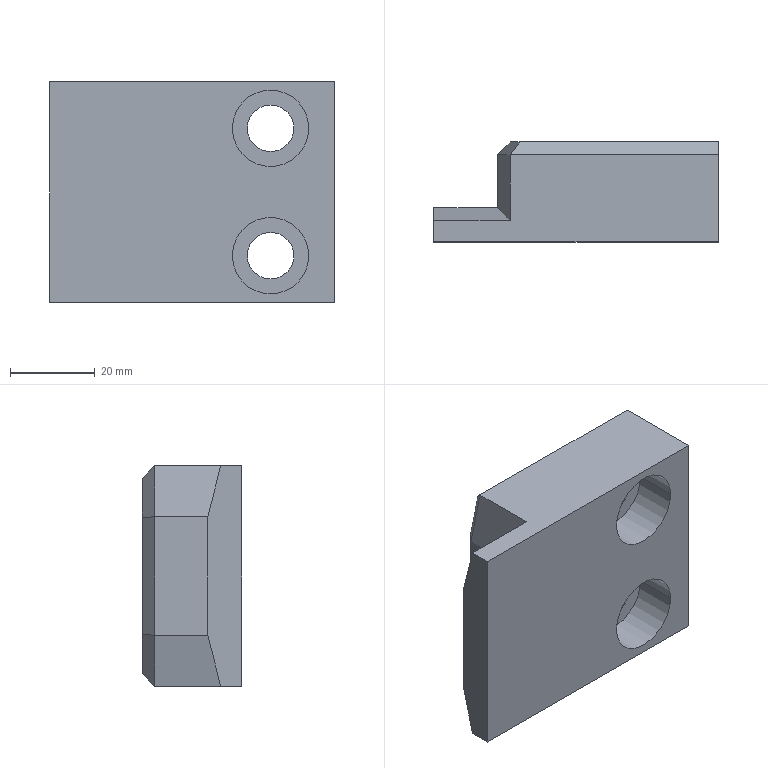Component | SolidWorks | EE8-214-_-_O-2 | 1 solid | 27 faces | box 67 x 23.5 x 52 mm | volume 60297 mm3 | plane 19 | cylinder 8 | commonest cylinder face diameters 18 x4 11 x4
build123d program:
from build123d import *
from OCP.BRepFilletAPI import BRepFilletAPI_MakeChamfer

# Parameters (mm, degrees)
EXTRUDE1_DEPTH                                       = 26
CHAMFER1_SIZE                                        = 3
CHAMFER1_SIZE2                                       = 12
CHAMFER2_SIZE                                        = 12
CHAMFER2_SIZE2                                       = 3
CHAMFER3_SIZE                                        = 3
COUNTERBORE_FOR_M10_SOCKET_HEAD_CAP_SCRE_D           = 11
COUNTERBORE_FOR_M10_SOCKET_HEAD_CAP_SCRE_CBORE_D     = 18
COUNTERBORE_FOR_M10_SOCKET_HEAD_CAP_SCRE_CBORE_DEPTH = 10


with BuildPart() as part:
    # Sketch1 → Extrude1 (new, symmetric)
    with BuildSketch(Plane(origin=(0, 0, 0), x_dir=(0, 0, -1), z_dir=(1, 0, 0))):
        Polygon((0, 0), (0, 23.5), (-52, 23.5), (-52, 8), (-67, 8), (-67, 0), align=None)
    extrude(amount=EXTRUDE1_DEPTH, both=True)

    # Chamfer1
    chamfer1_edges = [part.edges().sort_by_distance(p)[0] for p in [
        (-26, 8, 59.5),
        (-26, 15.75, 52),
    ]]
    chamfer1_side = [part.faces().sort_by_distance(p)[0] for p in [
        (-26, 11.057, 28.996),
    ]]
    chamfer(chamfer1_edges, length=CHAMFER1_SIZE, length2=CHAMFER1_SIZE2, reference=chamfer1_side[0])

    # Chamfer2: one chamfer whose edges measure the first distance from different faces: ONE call of the kernel's chamfer builder (chamfer() names one face for all edges)
    chamfer2_edges_1 = [part.edges().sort_by_distance(p)[0] for p in [
        (26, 15.75, 52),
    ]]
    chamfer2_side_1 = [part.faces().sort_by_distance(p)[0] for p in [
        (6, 15.75, 52),
    ]]
    chamfer2_edges_2 = [part.edges().sort_by_distance(p)[0] for p in [
        (26, 8, 59.5),
    ]]
    chamfer2_side_2 = [part.faces().sort_by_distance(p)[0] for p in [
        (6, 8, 59.5),
    ]]
    chamfer2 = BRepFilletAPI_MakeChamfer(part.part.solid().wrapped)
    for e in chamfer2_edges_1:
        chamfer2.Add(CHAMFER2_SIZE, CHAMFER2_SIZE2, e.wrapped, chamfer2_side_1[0].wrapped)  # the first distance lies on this face
    for e in chamfer2_edges_2:
        chamfer2.Add(CHAMFER2_SIZE, CHAMFER2_SIZE2, e.wrapped, chamfer2_side_2[0].wrapped)  # the first distance lies on this face
    add(Compound.cast(chamfer2.Shape()), mode=Mode.REPLACE)

    # Chamfer3
    chamfer3_edges = [part.edges().sort_by_distance(p)[0] for p in [
        (26, 23.5, 24.5),
        (-20, 23.5, 50.5),
        (0, 23.5, 52),
        (20, 23.5, 50.5),
        (-26, 23.5, 24.5),
    ]]
    chamfer(chamfer3_edges, length=CHAMFER3_SIZE)

    # Counterbore for M10 Socket Head Cap Scre (through all)
    with Locations(Plane.XZ):
        with Locations((15, 15), (-15, 15)):
            CounterBoreHole(COUNTERBORE_FOR_M10_SOCKET_HEAD_CAP_SCRE_D / 2, COUNTERBORE_FOR_M10_SOCKET_HEAD_CAP_SCRE_CBORE_D / 2, COUNTERBORE_FOR_M10_SOCKET_HEAD_CAP_SCRE_CBORE_DEPTH)


solid = part.part

# Placed as in the assembly
solid = solid.moved(Location((15, -23.5, -230), (0, -90, 0)))
STEP:
#1=CARTESIAN_POINT('',(-0.3543,-0.5315,-9.646));
#2=VERTEX_POINT('',#1);
#3=CARTESIAN_POINT('',(0.3543,-0.5315,-9.646));
#4=VERTEX_POINT('',#3);
#5=CARTESIAN_POINT('',(-0.,-0.5315,-9.646));
#6=DIRECTION('',(0.,-1.,0.));
#7=DIRECTION('',(1.,0.,-0.));
#8=AXIS2_PLACEMENT_3D('',#5,#6,#7);
#9=CIRCLE('',#8,0.3543);
#10=EDGE_CURVE('',#2,#4,#9,.T.);
#11=ORIENTED_EDGE('',*,*,#10,.F.);
#12=CARTESIAN_POINT('',(-0.3543,-0.9252,-9.646));
#13=VERTEX_POINT('',#12);
#14=CARTESIAN_POINT('',(-0.3543,-0.9252,-9.646));
#15=DIRECTION('',(0.,-1.,0.));
#16=VECTOR('',#15,39.37);
#17=LINE('',#14,#16);
#18=EDGE_CURVE('',#2,#13,#17,.T.);
#19=ORIENTED_EDGE('',*,*,#18,.T.);
#20=CARTESIAN_POINT('',(0.3543,-0.9252,-9.646));
#21=VERTEX_POINT('',#20);
#22=CARTESIAN_POINT('',(-0.,-0.9252,-9.646));
#23=DIRECTION('',(0.,-1.,0.));
#24=DIRECTION('',(1.,0.,-0.));
#25=AXIS2_PLACEMENT_3D('',#22,#23,#24);
#26=CIRCLE('',#25,0.3543);
#27=EDGE_CURVE('',#13,#21,#26,.T.);
#28=ORIENTED_EDGE('',*,*,#27,.T.);
#29=CARTESIAN_POINT('',(0.3543,-0.9252,-9.646));
#30=DIRECTION('',(0.,-1.,0.));
#31=VECTOR('',#30,39.37);
#32=LINE('',#29,#31);
#33=EDGE_CURVE('',#4,#21,#32,.T.);
#34=ORIENTED_EDGE('',*,*,#33,.F.);
#35=EDGE_LOOP('',(#11,#19,#28,#34));
#36=FACE_OUTER_BOUND('',#35,.T.);
#37=CARTESIAN_POINT('',(-0.,-0.9252,-9.646));
#38=DIRECTION('',(0.,-1.,0.));
#39=DIRECTION('',(1.,0.,-0.));
#40=AXIS2_PLACEMENT_3D('',#37,#38,#39);
#41=CYLINDRICAL_SURFACE('',#40,0.3543);
#42=ADVANCED_FACE('',(#36),#41,.F.);
#43=CARTESIAN_POINT('',(-0.2165,0.,-9.646));
#44=VERTEX_POINT('',#43);
#45=CARTESIAN_POINT('',(0.2165,0.,-9.646));
#46=VERTEX_POINT('',#45);
#47=CARTESIAN_POINT('',(-0.,0.,-9.646));
#48=DIRECTION('',(0.,-1.,0.));
#49=DIRECTION('',(1.,0.,-0.));
#50=AXIS2_PLACEMENT_3D('',#47,#48,#49);
#51=CIRCLE('',#50,0.2165);
#52=EDGE_CURVE('',#44,#46,#51,.T.);
#53=ORIENTED_EDGE('',*,*,#52,.F.);
#54=CARTESIAN_POINT('',(-0.2165,-0.5315,-9.646));
#55=VERTEX_POINT('',#54);
#56=CARTESIAN_POINT('',(-0.2165,-0.9252,-9.646));
#57=DIRECTION('',(0.,-1.,0.));
#58=VECTOR('',#57,39.37);
#59=LINE('',#56,#58);
#60=EDGE_CURVE('',#44,#55,#59,.T.);
#61=ORIENTED_EDGE('',*,*,#60,.T.);
#62=CARTESIAN_POINT('',(0.2165,-0.5315,-9.646));
#63=VERTEX_POINT('',#62);
#64=CARTESIAN_POINT('',(-0.,-0.5315,-9.646));
#65=DIRECTION('',(0.,-1.,0.));
#66=DIRECTION('',(1.,0.,-0.));
#67=AXIS2_PLACEMENT_3D('',#64,#65,#66);
#68=CIRCLE('',#67,0.2165);
#69=EDGE_CURVE('',#55,#63,#68,.T.);
#70=ORIENTED_EDGE('',*,*,#69,.T.);
#71=CARTESIAN_POINT('',(0.2165,-0.9252,-9.646));
#72=DIRECTION('',(0.,-1.,0.));
#73=VECTOR('',#72,39.37);
#74=LINE('',#71,#73);
#75=EDGE_CURVE('',#46,#63,#74,.T.);
#76=ORIENTED_EDGE('',*,*,#75,.F.);
#77=EDGE_LOOP('',(#53,#61,#70,#76));
#78=FACE_OUTER_BOUND('',#77,.T.);
#79=CARTESIAN_POINT('',(-0.,-0.9252,-9.646));
#80=DIRECTION('',(0.,-1.,0.));
#81=DIRECTION('',(1.,0.,-0.));
#82=AXIS2_PLACEMENT_3D('',#79,#80,#81);
#83=CYLINDRICAL_SURFACE('',#82,0.2165);
#84=ADVANCED_FACE('',(#78),#83,.F.);
#85=CARTESIAN_POINT('',(-0.3543,-0.5315,-8.465));
#86=VERTEX_POINT('',#85);
#87=CARTESIAN_POINT('',(0.3543,-0.5315,-8.465));
#88=VERTEX_POINT('',#87);
#89=CARTESIAN_POINT('',(-0.,-0.5315,-8.465));
#90=DIRECTION('',(0.,-1.,0.));
#91=DIRECTION('',(1.,0.,-0.));
#92=AXIS2_PLACEMENT_3D('',#89,#90,#91);
#93=CIRCLE('',#92,0.3543);
#94=EDGE_CURVE('',#86,#88,#93,.T.);
#95=ORIENTED_EDGE('',*,*,#94,.F.);
#96=CARTESIAN_POINT('',(-0.3543,-0.9252,-8.465));
#97=VERTEX_POINT('',#96);
#98=CARTESIAN_POINT('',(-0.3543,-0.9252,-8.465));
#99=DIRECTION('',(0.,-1.,0.));
#100=VECTOR('',#99,39.37);
#101=LINE('',#98,#100);
#102=EDGE_CURVE('',#86,#97,#101,.T.);
#103=ORIENTED_EDGE('',*,*,#102,.T.);
#104=CARTESIAN_POINT('',(0.3543,-0.9252,-8.465));
#105=VERTEX_POINT('',#104);
#106=CARTESIAN_POINT('',(-0.,-0.9252,-8.465));
#107=DIRECTION('',(0.,-1.,0.));
#108=DIRECTION('',(1.,0.,-0.));
#109=AXIS2_PLACEMENT_3D('',#106,#107,#108);
#110=CIRCLE('',#109,0.3543);
#111=EDGE_CURVE('',#97,#105,#110,.T.);
#112=ORIENTED_EDGE('',*,*,#111,.T.);
#113=CARTESIAN_POINT('',(0.3543,-0.9252,-8.465));
#114=DIRECTION('',(0.,-1.,0.));
#115=VECTOR('',#114,39.37);
#116=LINE('',#113,#115);
#117=EDGE_CURVE('',#88,#105,#116,.T.);
#118=ORIENTED_EDGE('',*,*,#117,.F.);
#119=EDGE_LOOP('',(#95,#103,#112,#118));
#120=FACE_OUTER_BOUND('',#119,.T.);
#121=CARTESIAN_POINT('',(-0.,-0.9252,-8.465));
#122=DIRECTION('',(0.,-1.,0.));
#123=DIRECTION('',(1.,0.,-0.));
#124=AXIS2_PLACEMENT_3D('',#121,#122,#123);
#125=CYLINDRICAL_SURFACE('',#124,0.3543);
#126=ADVANCED_FACE('',(#120),#125,.F.);
#127=CARTESIAN_POINT('',(-0.2165,0.,-8.465));
#128=VERTEX_POINT('',#127);
#129=CARTESIAN_POINT('',(0.2165,0.,-8.465));
#130=VERTEX_POINT('',#129);
#131=CARTESIAN_POINT('',(-0.,0.,-8.465));
#132=DIRECTION('',(0.,-1.,0.));
#133=DIRECTION('',(1.,0.,-0.));
#134=AXIS2_PLACEMENT_3D('',#131,#132,#133);
#135=CIRCLE('',#134,0.2165);
#136=EDGE_CURVE('',#128,#130,#135,.T.);
#137=ORIENTED_EDGE('',*,*,#136,.F.);
#138=CARTESIAN_POINT('',(-0.2165,-0.5315,-8.465));
#139=VERTEX_POINT('',#138);
#140=CARTESIAN_POINT('',(-0.2165,-0.9252,-8.465));
#141=DIRECTION('',(0.,-1.,0.));
#142=VECTOR('',#141,39.37);
#143=LINE('',#140,#142);
#144=EDGE_CURVE('',#128,#139,#143,.T.);
#145=ORIENTED_EDGE('',*,*,#144,.T.);
#146=CARTESIAN_POINT('',(0.2165,-0.5315,-8.465));
#147=VERTEX_POINT('',#146);
#148=CARTESIAN_POINT('',(-0.,-0.5315,-8.465));
#149=DIRECTION('',(0.,-1.,0.));
#150=DIRECTION('',(1.,0.,-0.));
#151=AXIS2_PLACEMENT_3D('',#148,#149,#150);
#152=CIRCLE('',#151,0.2165);
#153=EDGE_CURVE('',#139,#147,#152,.T.);
#154=ORIENTED_EDGE('',*,*,#153,.T.);
#155=CARTESIAN_POINT('',(0.2165,-0.9252,-8.465));
#156=DIRECTION('',(0.,-1.,0.));
#157=VECTOR('',#156,39.37);
#158=LINE('',#155,#157);
#159=EDGE_CURVE('',#130,#147,#158,.T.);
#160=ORIENTED_EDGE('',*,*,#159,.F.);
#161=EDGE_LOOP('',(#137,#145,#154,#160));
#162=FACE_OUTER_BOUND('',#161,.T.);
#163=CARTESIAN_POINT('',(-0.,-0.9252,-8.465));
#164=DIRECTION('',(0.,-1.,0.));
#165=DIRECTION('',(1.,0.,-0.));
#166=AXIS2_PLACEMENT_3D('',#163,#164,#165);
#167=CYLINDRICAL_SURFACE('',#166,0.2165);
#168=ADVANCED_FACE('',(#162),#167,.F.);
#169=CARTESIAN_POINT('',(-0.,-0.9252,-9.646));
#170=DIRECTION('',(0.,-1.,0.));
#171=DIRECTION('',(1.,0.,-0.));
#172=AXIS2_PLACEMENT_3D('',#169,#170,#171);
#173=CIRCLE('',#172,0.3543);
#174=EDGE_CURVE('',#21,#13,#173,.T.);
#175=ORIENTED_EDGE('',*,*,#174,.F.);
#176=ORIENTED_EDGE('',*,*,#27,.F.);
#177=EDGE_LOOP('',(#175,#176));
#178=FACE_BOUND('',#177,.T.);
#179=CARTESIAN_POINT('',(-2.047,-0.9252,-10.079));
#180=VERTEX_POINT('',#179);
#181=CARTESIAN_POINT('',(0.5906,-0.9252,-10.079));
#182=VERTEX_POINT('',#181);
#183=CARTESIAN_POINT('',(-2.047,-0.9252,-10.079));
#184=DIRECTION('',(1.,0.,-0.));
#185=VECTOR('',#184,39.37);
#186=LINE('',#183,#185);
#187=EDGE_CURVE('',#180,#182,#186,.T.);
#188=ORIENTED_EDGE('',*,*,#187,.T.);
#189=CARTESIAN_POINT('',(0.5906,-0.9252,-8.031));
#190=VERTEX_POINT('',#189);
#191=CARTESIAN_POINT('',(0.5906,-0.9252,-8.031));
#192=DIRECTION('',(-0.,0.,-1.));
#193=VECTOR('',#192,39.37);
#194=LINE('',#191,#193);
#195=EDGE_CURVE('',#190,#182,#194,.T.);
#196=ORIENTED_EDGE('',*,*,#195,.F.);
#197=CARTESIAN_POINT('',(-2.047,-0.9252,-8.031));
#198=VERTEX_POINT('',#197);
#199=CARTESIAN_POINT('',(-2.047,-0.9252,-8.031));
#200=DIRECTION('',(1.,0.,-0.));
#201=VECTOR('',#200,39.37);
#202=LINE('',#199,#201);
#203=EDGE_CURVE('',#198,#190,#202,.T.);
#204=ORIENTED_EDGE('',*,*,#203,.F.);
#205=CARTESIAN_POINT('',(-2.047,-0.9252,-8.031));
#206=DIRECTION('',(-0.,0.,-1.));
#207=VECTOR('',#206,39.37);
#208=LINE('',#205,#207);
#209=EDGE_CURVE('',#198,#180,#208,.T.);
#210=ORIENTED_EDGE('',*,*,#209,.T.);
#211=EDGE_LOOP('',(#188,#196,#204,#210));
#212=FACE_OUTER_BOUND('',#211,.T.);
#213=CARTESIAN_POINT('',(-0.,-0.9252,-8.465));
#214=DIRECTION('',(0.,-1.,0.));
#215=DIRECTION('',(1.,0.,-0.));
#216=AXIS2_PLACEMENT_3D('',#213,#214,#215);
#217=CIRCLE('',#216,0.3543);
#218=EDGE_CURVE('',#105,#97,#217,.T.);
#219=ORIENTED_EDGE('',*,*,#218,.F.);
#220=ORIENTED_EDGE('',*,*,#111,.F.);
#221=EDGE_LOOP('',(#219,#220));
#222=FACE_BOUND('',#221,.T.);
#223=CARTESIAN_POINT('',(-2.047,-0.9252,-8.031));
#224=DIRECTION('',(0.,1.,0.));
#225=DIRECTION('',(-1.,0.,0.));
#226=AXIS2_PLACEMENT_3D('',#223,#224,#225);
#227=PLANE('',#226);
#228=ADVANCED_FACE('',(#178,#212,#222),#227,.F.);
#229=CARTESIAN_POINT('',(0.5906,-0.1181,-10.079));
#230=VERTEX_POINT('',#229);
#231=CARTESIAN_POINT('',(0.5906,-0.9252,-10.079));
#232=DIRECTION('',(0.,1.,0.));
#233=VECTOR('',#232,39.37);
#234=LINE('',#231,#233);
#235=EDGE_CURVE('',#182,#230,#234,.T.);
#236=ORIENTED_EDGE('',*,*,#235,.T.);
#237=CARTESIAN_POINT('',(0.5906,0.,-9.961));
#238=VERTEX_POINT('',#237);
#239=CARTESIAN_POINT('',(0.5906,0.,-9.961));
#240=DIRECTION('',(0.,0.7071,0.7071));
#241=VECTOR('',#240,39.37);
#242=LINE('',#239,#241);
#243=EDGE_CURVE('',#230,#238,#242,.T.);
#244=ORIENTED_EDGE('',*,*,#243,.T.);
#245=CARTESIAN_POINT('',(0.5906,0.,-8.15));
#246=VERTEX_POINT('',#245);
#247=CARTESIAN_POINT('',(0.5906,0.,-8.031));
#248=DIRECTION('',(-0.,0.,-1.));
#249=VECTOR('',#248,39.37);
#250=LINE('',#247,#249);
#251=EDGE_CURVE('',#246,#238,#250,.T.);
#252=ORIENTED_EDGE('',*,*,#251,.F.);
#253=CARTESIAN_POINT('',(0.5906,-0.1181,-8.031));
#254=VERTEX_POINT('',#253);
#255=CARTESIAN_POINT('',(0.5906,-0.1181,-8.031));
#256=DIRECTION('',(0.,-0.7071,0.7071));
#257=VECTOR('',#256,39.37);
#258=LINE('',#255,#257);
#259=EDGE_CURVE('',#246,#254,#258,.T.);
#260=ORIENTED_EDGE('',*,*,#259,.T.);
#261=CARTESIAN_POINT('',(0.5906,-0.9252,-8.031));
#262=DIRECTION('',(0.,1.,0.));
#263=VECTOR('',#262,39.37);
#264=LINE('',#261,#263);
#265=EDGE_CURVE('',#190,#254,#264,.T.);
#266=ORIENTED_EDGE('',*,*,#265,.F.);
#267=ORIENTED_EDGE('',*,*,#195,.T.);
#268=EDGE_LOOP('',(#236,#244,#252,#260,#266,#267));
#269=FACE_OUTER_BOUND('',#268,.T.);
#270=CARTESIAN_POINT('',(0.5906,-0.9252,-8.031));
#271=DIRECTION('',(-1.,0.,0.));
#272=DIRECTION('',(0.,0.,1.));
#273=AXIS2_PLACEMENT_3D('',#270,#271,#272);
#274=PLANE('',#273);
#275=ADVANCED_FACE('',(#269),#274,.F.);
#276=CARTESIAN_POINT('',(-0.,0.,-9.646));
#277=DIRECTION('',(0.,-1.,0.));
#278=DIRECTION('',(1.,0.,-0.));
#279=AXIS2_PLACEMENT_3D('',#276,#277,#278);
#280=CIRCLE('',#279,0.2165);
#281=EDGE_CURVE('',#46,#44,#280,.T.);
#282=ORIENTED_EDGE('',*,*,#281,.T.);
#283=ORIENTED_EDGE('',*,*,#52,.T.);
#284=EDGE_LOOP('',(#282,#283));
#285=FACE_BOUND('',#284,.T.);
#286=CARTESIAN_POINT('',(-0.,0.,-8.465));
#287=DIRECTION('',(0.,-1.,0.));
#288=DIRECTION('',(1.,0.,-0.));
#289=AXIS2_PLACEMENT_3D('',#286,#287,#288);
#290=CIRCLE('',#289,0.2165);
#291=EDGE_CURVE('',#130,#128,#290,.T.);
#292=ORIENTED_EDGE('',*,*,#291,.T.);
#293=ORIENTED_EDGE('',*,*,#136,.T.);
#294=EDGE_LOOP('',(#292,#293));
#295=FACE_BOUND('',#294,.T.);
#296=ORIENTED_EDGE('',*,*,#251,.T.);
#297=CARTESIAN_POINT('',(-1.246,-0.,-9.961));
#298=VERTEX_POINT('',#297);
#299=CARTESIAN_POINT('',(0.5906,0.,-9.961));
#300=DIRECTION('',(-1.,-0.,0.));
#301=VECTOR('',#300,39.37);
#302=LINE('',#299,#301);
#303=EDGE_CURVE('',#238,#298,#302,.T.);
#304=ORIENTED_EDGE('',*,*,#303,.T.);
#305=CARTESIAN_POINT('',(-1.339,-0.,-9.592));
#306=VERTEX_POINT('',#305);
#307=CARTESIAN_POINT('',(-1.342,-0.,-9.578));
#308=DIRECTION('',(-0.2425,-0.,0.9701));
#309=VECTOR('',#308,39.37);
#310=LINE('',#307,#309);
#311=EDGE_CURVE('',#298,#306,#310,.T.);
#312=ORIENTED_EDGE('',*,*,#311,.T.);
#313=CARTESIAN_POINT('',(-1.339,-0.,-8.518));
#314=VERTEX_POINT('',#313);
#315=CARTESIAN_POINT('',(-1.339,-0.,-8.031));
#316=DIRECTION('',(0.,0.,1.));
#317=VECTOR('',#316,39.37);
#318=LINE('',#315,#317);
#319=EDGE_CURVE('',#306,#314,#318,.T.);
#320=ORIENTED_EDGE('',*,*,#319,.T.);
#321=CARTESIAN_POINT('',(-1.246,-0.,-8.15));
#322=VERTEX_POINT('',#321);
#323=CARTESIAN_POINT('',(-1.224,-0.,-8.06));
#324=DIRECTION('',(0.2425,0.,0.9701));
#325=VECTOR('',#324,39.37);
#326=LINE('',#323,#325);
#327=EDGE_CURVE('',#314,#322,#326,.T.);
#328=ORIENTED_EDGE('',*,*,#327,.T.);
#329=CARTESIAN_POINT('',(0.5906,0.,-8.15));
#330=DIRECTION('',(1.,0.,-0.));
#331=VECTOR('',#330,39.37);
#332=LINE('',#329,#331);
#333=EDGE_CURVE('',#322,#246,#332,.T.);
#334=ORIENTED_EDGE('',*,*,#333,.T.);
#335=EDGE_LOOP('',(#296,#304,#312,#320,#328,#334));
#336=FACE_OUTER_BOUND('',#335,.T.);
#337=CARTESIAN_POINT('',(0.5906,0.,-8.031));
#338=DIRECTION('',(0.,-1.,-0.));
#339=DIRECTION('',(1.,0.,-0.));
#340=AXIS2_PLACEMENT_3D('',#337,#338,#339);
#341=PLANE('',#340);
#342=ADVANCED_FACE('',(#285,#295,#336),#341,.F.);
#343=CARTESIAN_POINT('',(-1.457,-0.6102,-8.504));
#344=VERTEX_POINT('',#343);
#345=CARTESIAN_POINT('',(-1.457,-0.1181,-8.504));
#346=VERTEX_POINT('',#345);
#347=CARTESIAN_POINT('',(-1.457,-0.,-8.504));
#348=DIRECTION('',(-0.,1.,0.));
#349=VECTOR('',#348,39.37);
#350=LINE('',#347,#349);
#351=EDGE_CURVE('',#344,#346,#350,.T.);
#352=ORIENTED_EDGE('',*,*,#351,.T.);
#353=CARTESIAN_POINT('',(-1.457,-0.1181,-9.606));
#354=VERTEX_POINT('',#353);
#355=CARTESIAN_POINT('',(-1.457,-0.1181,-8.031));
#356=DIRECTION('',(-0.,0.,-1.));
#357=VECTOR('',#356,39.37);
#358=LINE('',#355,#357);
#359=EDGE_CURVE('',#346,#354,#358,.T.);
#360=ORIENTED_EDGE('',*,*,#359,.T.);
#361=CARTESIAN_POINT('',(-1.457,-0.6102,-9.606));
#362=VERTEX_POINT('',#361);
#363=CARTESIAN_POINT('',(-1.457,-0.,-9.606));
#364=DIRECTION('',(0.,-1.,-0.));
#365=VECTOR('',#364,39.37);
#366=LINE('',#363,#365);
#367=EDGE_CURVE('',#354,#362,#366,.T.);
#368=ORIENTED_EDGE('',*,*,#367,.T.);
#369=CARTESIAN_POINT('',(-1.457,-0.6102,-8.031));
#370=DIRECTION('',(-0.,0.,-1.));
#371=VECTOR('',#370,39.37);
#372=LINE('',#369,#371);
#373=EDGE_CURVE('',#344,#362,#372,.T.);
#374=ORIENTED_EDGE('',*,*,#373,.F.);
#375=EDGE_LOOP('',(#352,#360,#368,#374));
#376=FACE_OUTER_BOUND('',#375,.T.);
#377=CARTESIAN_POINT('',(-1.457,-0.,-8.031));
#378=DIRECTION('',(1.,0.,-0.));
#379=DIRECTION('',(-0.,1.,0.));
#380=AXIS2_PLACEMENT_3D('',#377,#378,#379);
#381=PLANE('',#380);
#382=ADVANCED_FACE('',(#376),#381,.F.);
#383=CARTESIAN_POINT('',(-2.047,-0.6102,-8.504));
#384=VERTEX_POINT('',#383);
#385=CARTESIAN_POINT('',(-2.047,-0.6102,-9.606));
#386=VERTEX_POINT('',#385);
#387=CARTESIAN_POINT('',(-2.047,-0.6102,-8.031));
#388=DIRECTION('',(-0.,0.,-1.));
#389=VECTOR('',#388,39.37);
#390=LINE('',#387,#389);
#391=EDGE_CURVE('',#384,#386,#390,.T.);
#392=ORIENTED_EDGE('',*,*,#391,.F.);
#393=CARTESIAN_POINT('',(-1.457,-0.6102,-8.504));
#394=DIRECTION('',(1.,0.,-0.));
#395=VECTOR('',#394,39.37);
#396=LINE('',#393,#395);
#397=EDGE_CURVE('',#384,#344,#396,.T.);
#398=ORIENTED_EDGE('',*,*,#397,.T.);
#399=ORIENTED_EDGE('',*,*,#373,.T.);
#400=CARTESIAN_POINT('',(-1.457,-0.6102,-9.606));
#401=DIRECTION('',(-1.,-0.,0.));
#402=VECTOR('',#401,39.37);
#403=LINE('',#400,#402);
#404=EDGE_CURVE('',#362,#386,#403,.T.);
#405=ORIENTED_EDGE('',*,*,#404,.T.);
#406=EDGE_LOOP('',(#392,#398,#399,#405));
#407=FACE_OUTER_BOUND('',#406,.T.);
#408=CARTESIAN_POINT('',(-1.457,-0.6102,-8.031));
#409=DIRECTION('',(0.,-1.,-0.));
#410=DIRECTION('',(1.,0.,-0.));
#411=AXIS2_PLACEMENT_3D('',#408,#409,#410);
#412=PLANE('',#411);
#413=ADVANCED_FACE('',(#407),#412,.F.);
#414=CARTESIAN_POINT('',(-2.047,-0.7283,-8.031));
#415=VERTEX_POINT('',#414);
#416=CARTESIAN_POINT('',(-2.047,-0.6102,-8.031));
#417=DIRECTION('',(0.,-1.,0.));
#418=VECTOR('',#417,39.37);
#419=LINE('',#416,#418);
#420=EDGE_CURVE('',#415,#198,#419,.T.);
#421=ORIENTED_EDGE('',*,*,#420,.F.);
#422=CARTESIAN_POINT('',(-2.047,-0.7283,-8.031));
#423=DIRECTION('',(-0.,0.2425,-0.9701));
#424=VECTOR('',#423,39.37);
#425=LINE('',#422,#424);
#426=EDGE_CURVE('',#415,#384,#425,.T.);
#427=ORIENTED_EDGE('',*,*,#426,.T.);
#428=ORIENTED_EDGE('',*,*,#391,.T.);
#429=CARTESIAN_POINT('',(-2.047,-0.7283,-10.079));
#430=VERTEX_POINT('',#429);
#431=CARTESIAN_POINT('',(-2.047,-0.6102,-9.606));
#432=DIRECTION('',(-0.,-0.2425,-0.9701));
#433=VECTOR('',#432,39.37);
#434=LINE('',#431,#433);
#435=EDGE_CURVE('',#386,#430,#434,.T.);
#436=ORIENTED_EDGE('',*,*,#435,.T.);
#437=CARTESIAN_POINT('',(-2.047,-0.6102,-10.079));
#438=DIRECTION('',(0.,-1.,0.));
#439=VECTOR('',#438,39.37);
#440=LINE('',#437,#439);
#441=EDGE_CURVE('',#430,#180,#440,.T.);
#442=ORIENTED_EDGE('',*,*,#441,.T.);
#443=ORIENTED_EDGE('',*,*,#209,.F.);
#444=EDGE_LOOP('',(#421,#427,#428,#436,#442,#443));
#445=FACE_OUTER_BOUND('',#444,.T.);
#446=CARTESIAN_POINT('',(-2.047,-0.6102,-8.031));
#447=DIRECTION('',(1.,0.,-0.));
#448=DIRECTION('',(-0.,0.,-1.));
#449=AXIS2_PLACEMENT_3D('',#446,#447,#448);
#450=PLANE('',#449);
#451=ADVANCED_FACE('',(#445),#450,.F.);
#452=ORIENTED_EDGE('',*,*,#265,.T.);
#453=CARTESIAN_POINT('',(-1.339,-0.1181,-8.031));
#454=VERTEX_POINT('',#453);
#455=CARTESIAN_POINT('',(-1.339,-0.1181,-8.031));
#456=DIRECTION('',(-1.,-0.,0.));
#457=VECTOR('',#456,39.37);
#458=LINE('',#455,#457);
#459=EDGE_CURVE('',#254,#454,#458,.T.);
#460=ORIENTED_EDGE('',*,*,#459,.T.);
#461=CARTESIAN_POINT('',(-1.339,-0.7283,-8.031));
#462=VERTEX_POINT('',#461);
#463=CARTESIAN_POINT('',(-1.339,-0.6102,-8.031));
#464=DIRECTION('',(0.,-1.,-0.));
#465=VECTOR('',#464,39.37);
#466=LINE('',#463,#465);
#467=EDGE_CURVE('',#454,#462,#466,.T.);
#468=ORIENTED_EDGE('',*,*,#467,.T.);
#469=CARTESIAN_POINT('',(-2.047,-0.7283,-8.031));
#470=DIRECTION('',(-1.,-0.,0.));
#471=VECTOR('',#470,39.37);
#472=LINE('',#469,#471);
#473=EDGE_CURVE('',#462,#415,#472,.T.);
#474=ORIENTED_EDGE('',*,*,#473,.T.);
#475=ORIENTED_EDGE('',*,*,#420,.T.);
#476=ORIENTED_EDGE('',*,*,#203,.T.);
#477=EDGE_LOOP('',(#452,#460,#468,#474,#475,#476));
#478=FACE_OUTER_BOUND('',#477,.T.);
#479=CARTESIAN_POINT('',(0.5906,-0.9252,-8.031));
#480=DIRECTION('',(0.,0.,1.));
#481=DIRECTION('',(1.,0.,-0.));
#482=AXIS2_PLACEMENT_3D('',#479,#480,#481);
#483=PLANE('',#482);
#484=ADVANCED_FACE('',(#478),#483,.T.);
#485=CARTESIAN_POINT('',(-1.339,-0.7283,-10.079));
#486=VERTEX_POINT('',#485);
#487=CARTESIAN_POINT('',(-1.339,-0.1181,-10.079));
#488=VERTEX_POINT('',#487);
#489=CARTESIAN_POINT('',(-1.339,-0.9252,-10.079));
#490=DIRECTION('',(-0.,1.,0.));
#491=VECTOR('',#490,39.37);
#492=LINE('',#489,#491);
#493=EDGE_CURVE('',#486,#488,#492,.T.);
#494=ORIENTED_EDGE('',*,*,#493,.T.);
#495=CARTESIAN_POINT('',(0.5906,-0.1181,-10.079));
#496=DIRECTION('',(1.,0.,-0.));
#497=VECTOR('',#496,39.37);
#498=LINE('',#495,#497);
#499=EDGE_CURVE('',#488,#230,#498,.T.);
#500=ORIENTED_EDGE('',*,*,#499,.T.);
#501=ORIENTED_EDGE('',*,*,#235,.F.);
#502=ORIENTED_EDGE('',*,*,#187,.F.);
#503=ORIENTED_EDGE('',*,*,#441,.F.);
#504=CARTESIAN_POINT('',(0.5906,-0.7283,-10.079));
#505=DIRECTION('',(1.,0.,-0.));
#506=VECTOR('',#505,39.37);
#507=LINE('',#504,#506);
#508=EDGE_CURVE('',#430,#486,#507,.T.);
#509=ORIENTED_EDGE('',*,*,#508,.T.);
#510=EDGE_LOOP('',(#494,#500,#501,#502,#503,#509));
#511=FACE_OUTER_BOUND('',#510,.T.);
#512=CARTESIAN_POINT('',(0.5906,-0.9252,-10.079));
#513=DIRECTION('',(0.,0.,1.));
#514=DIRECTION('',(1.,0.,-0.));
#515=AXIS2_PLACEMENT_3D('',#512,#513,#514);
#516=PLANE('',#515);
#517=ADVANCED_FACE('',(#511),#516,.F.);
#518=ORIENTED_EDGE('',*,*,#435,.F.);
#519=ORIENTED_EDGE('',*,*,#404,.F.);
#520=CARTESIAN_POINT('',(-1.491,-0.5763,-9.471));
#521=DIRECTION('',(-0.2357,0.2357,0.9428));
#522=VECTOR('',#521,39.37);
#523=LINE('',#520,#522);
#524=EDGE_CURVE('',#486,#362,#523,.T.);
#525=ORIENTED_EDGE('',*,*,#524,.F.);
#526=ORIENTED_EDGE('',*,*,#508,.F.);
#527=EDGE_LOOP('',(#518,#519,#525,#526));
#528=FACE_OUTER_BOUND('',#527,.T.);
#529=CARTESIAN_POINT('',(-1.457,-0.6102,-9.606));
#530=DIRECTION('',(0.,-0.9701,0.2425));
#531=DIRECTION('',(0.,0.2425,0.9701));
#532=AXIS2_PLACEMENT_3D('',#529,#530,#531);
#533=PLANE('',#532);
#534=ADVANCED_FACE('',(#528),#533,.F.);
#535=ORIENTED_EDGE('',*,*,#367,.F.);
#536=CARTESIAN_POINT('',(-1.339,-0.1181,-10.079));
#537=DIRECTION('',(0.2425,0.,-0.9701));
#538=VECTOR('',#537,39.37);
#539=LINE('',#536,#538);
#540=EDGE_CURVE('',#354,#488,#539,.T.);
#541=ORIENTED_EDGE('',*,*,#540,.T.);
#542=ORIENTED_EDGE('',*,*,#493,.F.);
#543=ORIENTED_EDGE('',*,*,#524,.T.);
#544=EDGE_LOOP('',(#535,#541,#542,#543));
#545=FACE_OUTER_BOUND('',#544,.T.);
#546=CARTESIAN_POINT('',(-1.457,-0.,-9.606));
#547=DIRECTION('',(0.9701,0.,0.2425));
#548=DIRECTION('',(0.2425,0.,-0.9701));
#549=AXIS2_PLACEMENT_3D('',#546,#547,#548);
#550=PLANE('',#549);
#551=ADVANCED_FACE('',(#545),#550,.F.);
#552=ORIENTED_EDGE('',*,*,#426,.F.);
#553=ORIENTED_EDGE('',*,*,#473,.F.);
#554=CARTESIAN_POINT('',(-1.328,-0.7393,-7.988));
#555=DIRECTION('',(0.2357,-0.2357,0.9428));
#556=VECTOR('',#555,39.37);
#557=LINE('',#554,#556);
#558=EDGE_CURVE('',#344,#462,#557,.T.);
#559=ORIENTED_EDGE('',*,*,#558,.F.);
#560=ORIENTED_EDGE('',*,*,#397,.F.);
#561=EDGE_LOOP('',(#552,#553,#559,#560));
#562=FACE_OUTER_BOUND('',#561,.T.);
#563=CARTESIAN_POINT('',(0.5906,-0.7283,-8.031));
#564=DIRECTION('',(0.,0.9701,0.2425));
#565=DIRECTION('',(-0.,0.2425,-0.9701));
#566=AXIS2_PLACEMENT_3D('',#563,#564,#565);
#567=PLANE('',#566);
#568=ADVANCED_FACE('',(#562),#567,.T.);
#569=ORIENTED_EDGE('',*,*,#467,.F.);
#570=CARTESIAN_POINT('',(-1.457,-0.1181,-8.504));
#571=DIRECTION('',(-0.2425,-0.,-0.9701));
#572=VECTOR('',#571,39.37);
#573=LINE('',#570,#572);
#574=EDGE_CURVE('',#454,#346,#573,.T.);
#575=ORIENTED_EDGE('',*,*,#574,.T.);
#576=ORIENTED_EDGE('',*,*,#351,.F.);
#577=ORIENTED_EDGE('',*,*,#558,.T.);
#578=EDGE_LOOP('',(#569,#575,#576,#577));
#579=FACE_OUTER_BOUND('',#578,.T.);
#580=CARTESIAN_POINT('',(-1.339,-0.9252,-8.031));
#581=DIRECTION('',(-0.9701,-0.,0.2425));
#582=DIRECTION('',(0.2425,0.,0.9701));
#583=AXIS2_PLACEMENT_3D('',#580,#581,#582);
#584=PLANE('',#583);
#585=ADVANCED_FACE('',(#579),#584,.T.);
#586=ORIENTED_EDGE('',*,*,#259,.F.);
#587=ORIENTED_EDGE('',*,*,#333,.F.);
#588=CARTESIAN_POINT('',(-1.377,-0.1676,-7.982));
#589=DIRECTION('',(0.4833,0.619,-0.619));
#590=VECTOR('',#589,39.37);
#591=LINE('',#588,#590);
#592=EDGE_CURVE('',#454,#322,#591,.T.);
#593=ORIENTED_EDGE('',*,*,#592,.F.);
#594=ORIENTED_EDGE('',*,*,#459,.F.);
#595=EDGE_LOOP('',(#586,#587,#593,#594));
#596=FACE_OUTER_BOUND('',#595,.T.);
#597=CARTESIAN_POINT('',(0.5906,-0.1181,-8.031));
#598=DIRECTION('',(0.,0.7071,0.7071));
#599=DIRECTION('',(-0.,0.7071,-0.7071));
#600=AXIS2_PLACEMENT_3D('',#597,#598,#599);
#601=PLANE('',#600);
#602=ADVANCED_FACE('',(#596),#601,.T.);
#603=ORIENTED_EDGE('',*,*,#592,.T.);
#604=ORIENTED_EDGE('',*,*,#327,.F.);
#605=CARTESIAN_POINT('',(-1.486,-0.147,-8.5));
#606=DIRECTION('',(0.7044,0.7044,-0.08672));
#607=VECTOR('',#606,39.37);
#608=LINE('',#605,#607);
#609=EDGE_CURVE('',#346,#314,#608,.T.);
#610=ORIENTED_EDGE('',*,*,#609,.F.);
#611=ORIENTED_EDGE('',*,*,#574,.F.);
#612=EDGE_LOOP('',(#603,#604,#610,#611));
#613=FACE_OUTER_BOUND('',#612,.T.);
#614=CARTESIAN_POINT('',(-1.111,-0.,-7.606));
#615=DIRECTION('',(-0.686,0.7071,0.1715));
#616=DIRECTION('',(-0.7177,-0.6963,0.));
#617=AXIS2_PLACEMENT_3D('',#614,#615,#616);
#618=PLANE('',#617);
#619=ADVANCED_FACE('',(#613),#618,.T.);
#620=ORIENTED_EDGE('',*,*,#609,.T.);
#621=ORIENTED_EDGE('',*,*,#319,.F.);
#622=CARTESIAN_POINT('',(-1.36,-0.02191,-9.594));
#623=DIRECTION('',(0.7044,0.7044,0.08672));
#624=VECTOR('',#623,39.37);
#625=LINE('',#622,#624);
#626=EDGE_CURVE('',#354,#306,#625,.T.);
#627=ORIENTED_EDGE('',*,*,#626,.F.);
#628=ORIENTED_EDGE('',*,*,#359,.F.);
#629=EDGE_LOOP('',(#620,#621,#627,#628));
#630=FACE_OUTER_BOUND('',#629,.T.);
#631=CARTESIAN_POINT('',(-1.457,-0.1181,-8.031));
#632=DIRECTION('',(0.7071,-0.7071,-0.));
#633=DIRECTION('',(0.7071,0.7071,-0.));
#634=AXIS2_PLACEMENT_3D('',#631,#632,#633);
#635=PLANE('',#634);
#636=ADVANCED_FACE('',(#630),#635,.F.);
#637=ORIENTED_EDGE('',*,*,#626,.T.);
#638=ORIENTED_EDGE('',*,*,#311,.F.);
#639=CARTESIAN_POINT('',(-0.9132,0.4267,-9.534));
#640=DIRECTION('',(0.4833,0.619,0.619));
#641=VECTOR('',#640,39.37);
#642=LINE('',#639,#641);
#643=EDGE_CURVE('',#488,#298,#642,.T.);
#644=ORIENTED_EDGE('',*,*,#643,.F.);
#645=ORIENTED_EDGE('',*,*,#540,.F.);
#646=EDGE_LOOP('',(#637,#638,#644,#645));
#647=FACE_OUTER_BOUND('',#646,.T.);
#648=CARTESIAN_POINT('',(-1.592,-0.,-8.577));
#649=DIRECTION('',(0.686,-0.7071,0.1715));
#650=DIRECTION('',(0.7177,0.6963,-0.));
#651=AXIS2_PLACEMENT_3D('',#648,#649,#650);
#652=PLANE('',#651);
#653=ADVANCED_FACE('',(#647),#652,.F.);
#654=ORIENTED_EDGE('',*,*,#243,.F.);
#655=ORIENTED_EDGE('',*,*,#499,.F.);
#656=ORIENTED_EDGE('',*,*,#643,.T.);
#657=ORIENTED_EDGE('',*,*,#303,.F.);
#658=EDGE_LOOP('',(#654,#655,#656,#657));
#659=FACE_OUTER_BOUND('',#658,.T.);
#660=CARTESIAN_POINT('',(0.5906,0.,-9.961));
#661=DIRECTION('',(0.,-0.7071,0.7071));
#662=DIRECTION('',(0.,0.7071,0.7071));
#663=AXIS2_PLACEMENT_3D('',#660,#661,#662);
#664=PLANE('',#663);
#665=ADVANCED_FACE('',(#659),#664,.F.);
#666=ORIENTED_EDGE('',*,*,#144,.F.);
#667=ORIENTED_EDGE('',*,*,#291,.F.);
#668=ORIENTED_EDGE('',*,*,#159,.T.);
#669=CARTESIAN_POINT('',(-0.,-0.5315,-8.465));
#670=DIRECTION('',(0.,-1.,0.));
#671=DIRECTION('',(1.,0.,-0.));
#672=AXIS2_PLACEMENT_3D('',#669,#670,#671);
#673=CIRCLE('',#672,0.2165);
#674=EDGE_CURVE('',#147,#139,#673,.T.);
#675=ORIENTED_EDGE('',*,*,#674,.T.);
#676=EDGE_LOOP('',(#666,#667,#668,#675));
#677=FACE_OUTER_BOUND('',#676,.T.);
#678=CARTESIAN_POINT('',(-0.,-0.9252,-8.465));
#679=DIRECTION('',(0.,-1.,0.));
#680=DIRECTION('',(1.,0.,-0.));
#681=AXIS2_PLACEMENT_3D('',#678,#679,#680);
#682=CYLINDRICAL_SURFACE('',#681,0.2165);
#683=ADVANCED_FACE('',(#677),#682,.F.);
#684=ORIENTED_EDGE('',*,*,#674,.F.);
#685=ORIENTED_EDGE('',*,*,#153,.F.);
#686=EDGE_LOOP('',(#684,#685));
#687=FACE_BOUND('',#686,.T.);
#688=CARTESIAN_POINT('',(-0.,-0.5315,-8.465));
#689=DIRECTION('',(0.,-1.,0.));
#690=DIRECTION('',(1.,0.,-0.));
#691=AXIS2_PLACEMENT_3D('',#688,#689,#690);
#692=CIRCLE('',#691,0.3543);
#693=EDGE_CURVE('',#88,#86,#692,.T.);
#694=ORIENTED_EDGE('',*,*,#693,.T.);
#695=ORIENTED_EDGE('',*,*,#94,.T.);
#696=EDGE_LOOP('',(#694,#695));
#697=FACE_OUTER_BOUND('',#696,.T.);
#698=CARTESIAN_POINT('',(-0.,-0.5315,-8.248));
#699=DIRECTION('',(0.,1.,0.));
#700=DIRECTION('',(-1.,0.,0.));
#701=AXIS2_PLACEMENT_3D('',#698,#699,#700);
#702=PLANE('',#701);
#703=ADVANCED_FACE('',(#687,#697),#702,.F.);
#704=ORIENTED_EDGE('',*,*,#102,.F.);
#705=ORIENTED_EDGE('',*,*,#693,.F.);
#706=ORIENTED_EDGE('',*,*,#117,.T.);
#707=ORIENTED_EDGE('',*,*,#218,.T.);
#708=EDGE_LOOP('',(#704,#705,#706,#707));
#709=FACE_OUTER_BOUND('',#708,.T.);
#710=CARTESIAN_POINT('',(-0.,-0.9252,-8.465));
#711=DIRECTION('',(0.,-1.,0.));
#712=DIRECTION('',(1.,0.,-0.));
#713=AXIS2_PLACEMENT_3D('',#710,#711,#712);
#714=CYLINDRICAL_SURFACE('',#713,0.3543);
#715=ADVANCED_FACE('',(#709),#714,.F.);
#716=ORIENTED_EDGE('',*,*,#60,.F.);
#717=ORIENTED_EDGE('',*,*,#281,.F.);
#718=ORIENTED_EDGE('',*,*,#75,.T.);
#719=CARTESIAN_POINT('',(-0.,-0.5315,-9.646));
#720=DIRECTION('',(0.,-1.,0.));
#721=DIRECTION('',(1.,0.,-0.));
#722=AXIS2_PLACEMENT_3D('',#719,#720,#721);
#723=CIRCLE('',#722,0.2165);
#724=EDGE_CURVE('',#63,#55,#723,.T.);
#725=ORIENTED_EDGE('',*,*,#724,.T.);
#726=EDGE_LOOP('',(#716,#717,#718,#725));
#727=FACE_OUTER_BOUND('',#726,.T.);
#728=CARTESIAN_POINT('',(-0.,-0.9252,-9.646));
#729=DIRECTION('',(0.,-1.,0.));
#730=DIRECTION('',(1.,0.,-0.));
#731=AXIS2_PLACEMENT_3D('',#728,#729,#730);
#732=CYLINDRICAL_SURFACE('',#731,0.2165);
#733=ADVANCED_FACE('',(#727),#732,.F.);
#734=ORIENTED_EDGE('',*,*,#724,.F.);
#735=ORIENTED_EDGE('',*,*,#69,.F.);
#736=EDGE_LOOP('',(#734,#735));
#737=FACE_BOUND('',#736,.T.);
#738=CARTESIAN_POINT('',(-0.,-0.5315,-9.646));
#739=DIRECTION('',(0.,-1.,0.));
#740=DIRECTION('',(1.,0.,-0.));
#741=AXIS2_PLACEMENT_3D('',#738,#739,#740);
#742=CIRCLE('',#741,0.3543);
#743=EDGE_CURVE('',#4,#2,#742,.T.);
#744=ORIENTED_EDGE('',*,*,#743,.T.);
#745=ORIENTED_EDGE('',*,*,#10,.T.);
#746=EDGE_LOOP('',(#744,#745));
#747=FACE_OUTER_BOUND('',#746,.T.);
#748=CARTESIAN_POINT('',(-0.,-0.5315,-9.429));
#749=DIRECTION('',(0.,1.,0.));
#750=DIRECTION('',(-1.,0.,0.));
#751=AXIS2_PLACEMENT_3D('',#748,#749,#750);
#752=PLANE('',#751);
#753=ADVANCED_FACE('',(#737,#747),#752,.F.);
#754=ORIENTED_EDGE('',*,*,#18,.F.);
#755=ORIENTED_EDGE('',*,*,#743,.F.);
#756=ORIENTED_EDGE('',*,*,#33,.T.);
#757=ORIENTED_EDGE('',*,*,#174,.T.);
#758=EDGE_LOOP('',(#754,#755,#756,#757));
#759=FACE_OUTER_BOUND('',#758,.T.);
#760=CARTESIAN_POINT('',(-0.,-0.9252,-9.646));
#761=DIRECTION('',(0.,-1.,0.));
#762=DIRECTION('',(1.,0.,-0.));
#763=AXIS2_PLACEMENT_3D('',#760,#761,#762);
#764=CYLINDRICAL_SURFACE('',#763,0.3543);
#765=ADVANCED_FACE('',(#759),#764,.F.);
#766=CLOSED_SHELL('',(#42,#84,#126,#168,#228,#275,#342,#382,#413,#451,#484,#517,#534,#551,#568,#585,#602,#619,#636,#653,#665,#683,#703,#715,#733,#753,#765));
#767=MANIFOLD_SOLID_BREP('',#766);
#768=CARTESIAN_POINT('',(0.,0.,0.));
#769=DIRECTION('',(0.,0.,1.));
#770=DIRECTION('',(1.,0.,0.));
#771=AXIS2_PLACEMENT_3D('',#768,#769,#770);
#772=(LENGTH_UNIT()NAMED_UNIT(*)SI_UNIT($,.METRE.));
#773=LENGTH_MEASURE_WITH_UNIT(LENGTH_MEASURE(0.0254),#772);
#774=DIMENSIONAL_EXPONENTS(1.,0.,0.,0.,0.,0.,0.);
#775=(CONVERSION_BASED_UNIT('',#773)LENGTH_UNIT()NAMED_UNIT(#774));
#776=UNCERTAINTY_MEASURE_WITH_UNIT(LENGTH_MEASURE(0.00001),#775,'','');
#777=(NAMED_UNIT(*)PLANE_ANGLE_UNIT()SI_UNIT($,.RADIAN.));
#778=(NAMED_UNIT(*)SI_UNIT($,.STERADIAN.)SOLID_ANGLE_UNIT());
#779=(GEOMETRIC_REPRESENTATION_CONTEXT(3)GLOBAL_UNCERTAINTY_ASSIGNED_CONTEXT((#776))GLOBAL_UNIT_ASSIGNED_CONTEXT((#775,#777,#778))REPRESENTATION_CONTEXT('',''));
#780=ADVANCED_BREP_SHAPE_REPRESENTATION('',(#767,#771),#779);
#781=COLOUR_RGB('',0.7922,0.8196,0.9333);
#782=FILL_AREA_STYLE_COLOUR('',#781);
#783=FILL_AREA_STYLE('',(#782));
#784=SURFACE_STYLE_FILL_AREA(#783);
#785=SURFACE_SIDE_STYLE('',(#784));
#786=SURFACE_STYLE_USAGE(.BOTH.,#785);
#787=PRESENTATION_STYLE_ASSIGNMENT((#786));
#788=STYLED_ITEM('',(#787),#767);
#789=(LENGTH_UNIT()NAMED_UNIT(*)SI_UNIT($,.METRE.));
#790=LENGTH_MEASURE_WITH_UNIT(LENGTH_MEASURE(0.0254),#789);
#791=DIMENSIONAL_EXPONENTS(1.,0.,0.,0.,0.,0.,0.);
#792=(CONVERSION_BASED_UNIT('',#790)LENGTH_UNIT()NAMED_UNIT(#791));
#793=UNCERTAINTY_MEASURE_WITH_UNIT(LENGTH_MEASURE(0.00001),#792,'','');
#794=(NAMED_UNIT(*)PLANE_ANGLE_UNIT()SI_UNIT($,.RADIAN.));
#795=(NAMED_UNIT(*)SI_UNIT($,.STERADIAN.)SOLID_ANGLE_UNIT());
#796=(GEOMETRIC_REPRESENTATION_CONTEXT(3)GLOBAL_UNCERTAINTY_ASSIGNED_CONTEXT((#793))GLOBAL_UNIT_ASSIGNED_CONTEXT((#792,#794,#795))REPRESENTATION_CONTEXT('',''));
#797=MECHANICAL_DESIGN_GEOMETRIC_PRESENTATION_REPRESENTATION('',(#788),#796);
#798=PRESENTATION_LAYER_ASSIGNMENT('','',(#788));